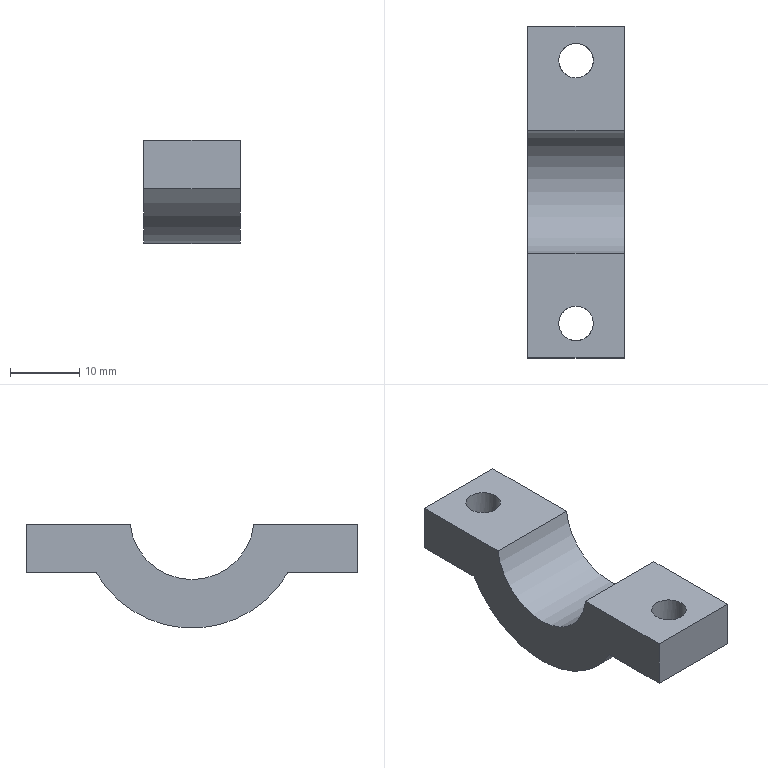Component | NX | LOWER_FIX_PLATE_2 | 1 solid | 16 faces | volume 4917 mm3 | plane 10 | cylinder 6 | commonest cylinder face diameters 5 x2 8 x2 32 x1 18 x1